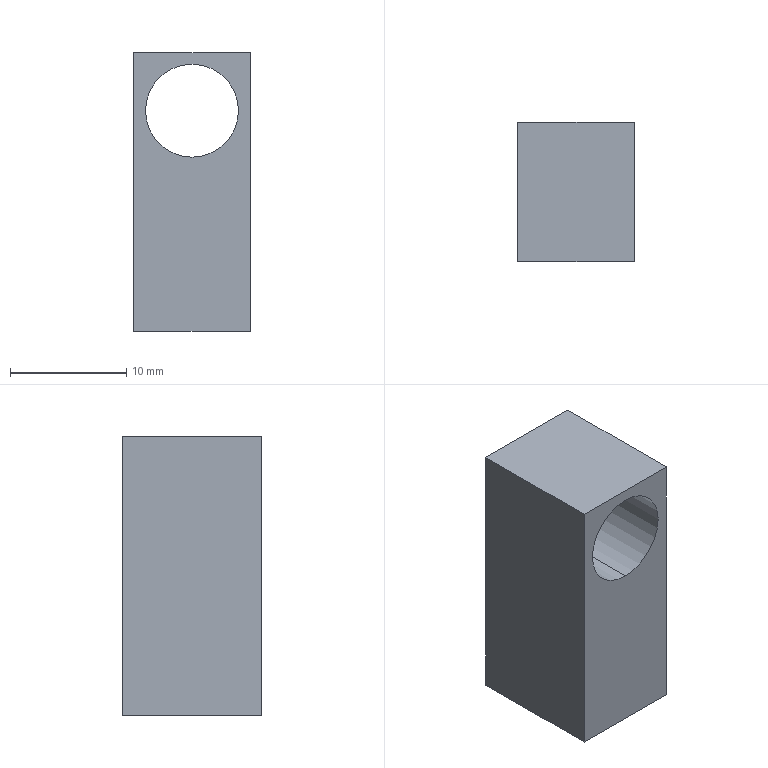Component | SolidWorks | HandlingMechanism-2_A0106-1 | 1 solid | 12 faces | box 10 x 12 x 24 mm | volume 2132 mm3 | plane 6 | cylinder 4 | cone 2 | commonest cylinder face diameters 8 x2 4.2 x2
build123d program:
from build123d import *

# Parameters (mm, degrees)
SKETCH1_W             = 12
SKETCH1_H             = 10
BOSS_EXTRUDE1_DEPTH   = 24
M5_TAPPED_HOLE1_D     = 4.2
M5_TAPPED_HOLE1_DEPTH = 10
M5_TAPPED_HOLE1_TIP   = 1.262
M8X1_0_TAPPED_HOLE1_D = 8


with BuildPart() as part:
    # Sketch1 → Boss-Extrude1 (new body)
    with BuildSketch(Plane.XY):
        Rectangle(SKETCH1_W, SKETCH1_H)
    extrude(amount=BOSS_EXTRUDE1_DEPTH)

    # M5 Tapped Hole1
    with Locations(Plane.XY.offset(24)):
        with Locations((0, 0)):
            Hole(M5_TAPPED_HOLE1_D / 2, depth=M5_TAPPED_HOLE1_DEPTH)
            with Locations((0, 0, -(M5_TAPPED_HOLE1_DEPTH + M5_TAPPED_HOLE1_TIP / 2))):  # 118° drill point
                Cone(0, M5_TAPPED_HOLE1_D / 2, M5_TAPPED_HOLE1_TIP, mode=Mode.SUBTRACT)

    # M8x1.0 Tapped Hole1 (through all)
    with Locations(Plane.ZY.offset(6)):
        with Locations((5, 0)):
            Hole(M8X1_0_TAPPED_HOLE1_D / 2)


solid = part.part

# Placed as in the assembly
solid = solid.moved(Location((80.881, 190.5, 157), (180, 0, -90)))
STEP:
#1=COLOUR_RGB('',0.7922,0.8196,0.9333);
#2=FILL_AREA_STYLE_COLOUR('',#1);
#3=FILL_AREA_STYLE('',(#2));
#4=SURFACE_STYLE_FILL_AREA(#3);
#5=SURFACE_SIDE_STYLE('',(#4));
#6=SURFACE_STYLE_USAGE(.BOTH.,#5);
#7=PRESENTATION_STYLE_ASSIGNMENT((#6));
#8=CARTESIAN_POINT('',(3.184,7.736,6.142));
#9=VERTEX_POINT('',#8);
#10=CARTESIAN_POINT('',(3.184,7.736,5.827));
#11=VERTEX_POINT('',#10);
#12=CARTESIAN_POINT('',(3.184,7.736,5.984));
#13=DIRECTION('',(-0.,-1.,0.));
#14=DIRECTION('',(0.,0.,-1.));
#15=AXIS2_PLACEMENT_3D('',#12,#13,#14);
#16=CIRCLE('',#15,0.1575);
#17=EDGE_CURVE('',#9,#11,#16,.T.);
#18=ORIENTED_EDGE('',*,*,#17,.F.);
#19=CARTESIAN_POINT('',(3.184,7.264,6.142));
#20=VERTEX_POINT('',#19);
#21=CARTESIAN_POINT('',(3.184,7.264,6.142));
#22=DIRECTION('',(-0.,-1.,0.));
#23=VECTOR('',#22,39.37);
#24=LINE('',#21,#23);
#25=EDGE_CURVE('',#9,#20,#24,.T.);
#26=ORIENTED_EDGE('',*,*,#25,.T.);
#27=CARTESIAN_POINT('',(3.184,7.264,5.827));
#28=VERTEX_POINT('',#27);
#29=CARTESIAN_POINT('',(3.184,7.264,5.984));
#30=DIRECTION('',(-0.,-1.,0.));
#31=DIRECTION('',(0.,0.,-1.));
#32=AXIS2_PLACEMENT_3D('',#29,#30,#31);
#33=CIRCLE('',#32,0.1575);
#34=EDGE_CURVE('',#20,#28,#33,.T.);
#35=ORIENTED_EDGE('',*,*,#34,.T.);
#36=CARTESIAN_POINT('',(3.184,7.264,5.827));
#37=DIRECTION('',(-0.,-1.,0.));
#38=VECTOR('',#37,39.37);
#39=LINE('',#36,#38);
#40=EDGE_CURVE('',#11,#28,#39,.T.);
#41=ORIENTED_EDGE('',*,*,#40,.F.);
#42=EDGE_LOOP('',(#18,#26,#35,#41));
#43=FACE_OUTER_BOUND('',#42,.T.);
#44=CARTESIAN_POINT('',(3.184,7.264,5.984));
#45=DIRECTION('',(-0.,-1.,0.));
#46=DIRECTION('',(0.,0.,-1.));
#47=AXIS2_PLACEMENT_3D('',#44,#45,#46);
#48=CYLINDRICAL_SURFACE('',#47,0.1575);
#49=ADVANCED_FACE('',(#43),#48,.F.);
#50=CARTESIAN_POINT('',(3.184,7.417,5.63));
#51=VERTEX_POINT('',#50);
#52=CARTESIAN_POINT('',(3.184,7.583,5.63));
#53=VERTEX_POINT('',#52);
#54=CARTESIAN_POINT('',(3.184,7.5,5.63));
#55=DIRECTION('',(0.,-0.,-1.));
#56=DIRECTION('',(0.,1.,0.));
#57=AXIS2_PLACEMENT_3D('',#54,#55,#56);
#58=CIRCLE('',#57,0.08268);
#59=EDGE_CURVE('',#51,#53,#58,.T.);
#60=ORIENTED_EDGE('',*,*,#59,.F.);
#61=CARTESIAN_POINT('',(3.184,7.417,5.236));
#62=VERTEX_POINT('',#61);
#63=CARTESIAN_POINT('',(3.184,7.417,5.236));
#64=DIRECTION('',(0.,-0.,-1.));
#65=VECTOR('',#64,39.37);
#66=LINE('',#63,#65);
#67=EDGE_CURVE('',#51,#62,#66,.T.);
#68=ORIENTED_EDGE('',*,*,#67,.T.);
#69=CARTESIAN_POINT('',(3.184,7.583,5.236));
#70=VERTEX_POINT('',#69);
#71=CARTESIAN_POINT('',(3.184,7.5,5.236));
#72=DIRECTION('',(0.,-0.,-1.));
#73=DIRECTION('',(0.,1.,0.));
#74=AXIS2_PLACEMENT_3D('',#71,#72,#73);
#75=CIRCLE('',#74,0.08268);
#76=EDGE_CURVE('',#62,#70,#75,.T.);
#77=ORIENTED_EDGE('',*,*,#76,.T.);
#78=CARTESIAN_POINT('',(3.184,7.583,5.236));
#79=DIRECTION('',(0.,-0.,-1.));
#80=VECTOR('',#79,39.37);
#81=LINE('',#78,#80);
#82=EDGE_CURVE('',#53,#70,#81,.T.);
#83=ORIENTED_EDGE('',*,*,#82,.F.);
#84=EDGE_LOOP('',(#60,#68,#77,#83));
#85=FACE_OUTER_BOUND('',#84,.T.);
#86=CARTESIAN_POINT('',(3.184,7.5,5.236));
#87=DIRECTION('',(0.,-0.,-1.));
#88=DIRECTION('',(0.,1.,0.));
#89=AXIS2_PLACEMENT_3D('',#86,#87,#88);
#90=CYLINDRICAL_SURFACE('',#89,0.08268);
#91=ADVANCED_FACE('',(#85),#90,.F.);
#92=CARTESIAN_POINT('',(3.184,7.5,5.68));
#93=VERTEX_POINT('',#92);
#94=CARTESIAN_POINT('',(3.184,7.583,5.63));
#95=DIRECTION('',(0.,0.8572,-0.515));
#96=VECTOR('',#95,39.37);
#97=LINE('',#94,#96);
#98=EDGE_CURVE('',#93,#53,#97,.T.);
#99=ORIENTED_EDGE('',*,*,#98,.F.);
#100=CARTESIAN_POINT('',(3.184,7.417,5.63));
#101=DIRECTION('',(0.,-0.8572,-0.515));
#102=VECTOR('',#101,39.37);
#103=LINE('',#100,#102);
#104=EDGE_CURVE('',#93,#51,#103,.T.);
#105=ORIENTED_EDGE('',*,*,#104,.T.);
#106=ORIENTED_EDGE('',*,*,#59,.T.);
#107=EDGE_LOOP('',(#99,#105,#106));
#108=FACE_OUTER_BOUND('',#107,.T.);
#109=CARTESIAN_POINT('',(3.184,7.5,5.63));
#110=DIRECTION('',(0.,-0.,-1.));
#111=DIRECTION('',(0.,1.,0.));
#112=AXIS2_PLACEMENT_3D('',#109,#110,#111);
#113=CONICAL_SURFACE('',#112,0.08268,1.03);
#114=ADVANCED_FACE('',(#108),#113,.F.);
#115=CARTESIAN_POINT('',(3.184,7.736,5.984));
#116=DIRECTION('',(-0.,-1.,0.));
#117=DIRECTION('',(0.,0.,-1.));
#118=AXIS2_PLACEMENT_3D('',#115,#116,#117);
#119=CIRCLE('',#118,0.1575);
#120=EDGE_CURVE('',#11,#9,#119,.T.);
#121=ORIENTED_EDGE('',*,*,#120,.T.);
#122=ORIENTED_EDGE('',*,*,#17,.T.);
#123=EDGE_LOOP('',(#121,#122));
#124=FACE_BOUND('',#123,.T.);
#125=CARTESIAN_POINT('',(2.987,7.736,6.181));
#126=VERTEX_POINT('',#125);
#127=CARTESIAN_POINT('',(3.381,7.736,6.181));
#128=VERTEX_POINT('',#127);
#129=CARTESIAN_POINT('',(3.381,7.736,6.181));
#130=DIRECTION('',(1.,-0.,0.));
#131=VECTOR('',#130,39.37);
#132=LINE('',#129,#131);
#133=EDGE_CURVE('',#126,#128,#132,.T.);
#134=ORIENTED_EDGE('',*,*,#133,.T.);
#135=CARTESIAN_POINT('',(3.381,7.736,5.236));
#136=VERTEX_POINT('',#135);
#137=CARTESIAN_POINT('',(3.381,7.736,5.236));
#138=DIRECTION('',(-0.,0.,1.));
#139=VECTOR('',#138,39.37);
#140=LINE('',#137,#139);
#141=EDGE_CURVE('',#136,#128,#140,.T.);
#142=ORIENTED_EDGE('',*,*,#141,.F.);
#143=CARTESIAN_POINT('',(2.987,7.736,5.236));
#144=VERTEX_POINT('',#143);
#145=CARTESIAN_POINT('',(3.381,7.736,5.236));
#146=DIRECTION('',(1.,-0.,0.));
#147=VECTOR('',#146,39.37);
#148=LINE('',#145,#147);
#149=EDGE_CURVE('',#144,#136,#148,.T.);
#150=ORIENTED_EDGE('',*,*,#149,.F.);
#151=CARTESIAN_POINT('',(2.987,7.736,5.236));
#152=DIRECTION('',(-0.,0.,1.));
#153=VECTOR('',#152,39.37);
#154=LINE('',#151,#153);
#155=EDGE_CURVE('',#144,#126,#154,.T.);
#156=ORIENTED_EDGE('',*,*,#155,.T.);
#157=EDGE_LOOP('',(#134,#142,#150,#156));
#158=FACE_OUTER_BOUND('',#157,.T.);
#159=CARTESIAN_POINT('',(3.381,7.736,5.236));
#160=DIRECTION('',(-0.,-1.,0.));
#161=DIRECTION('',(-1.,0.,-0.));
#162=AXIS2_PLACEMENT_3D('',#159,#160,#161);
#163=PLANE('',#162);
#164=ADVANCED_FACE('',(#124,#158),#163,.F.);
#165=CARTESIAN_POINT('',(3.381,7.264,6.181));
#166=VERTEX_POINT('',#165);
#167=CARTESIAN_POINT('',(3.381,7.264,6.181));
#168=DIRECTION('',(-0.,-1.,0.));
#169=VECTOR('',#168,39.37);
#170=LINE('',#167,#169);
#171=EDGE_CURVE('',#128,#166,#170,.T.);
#172=ORIENTED_EDGE('',*,*,#171,.T.);
#173=CARTESIAN_POINT('',(3.381,7.264,5.236));
#174=VERTEX_POINT('',#173);
#175=CARTESIAN_POINT('',(3.381,7.264,5.236));
#176=DIRECTION('',(-0.,0.,1.));
#177=VECTOR('',#176,39.37);
#178=LINE('',#175,#177);
#179=EDGE_CURVE('',#174,#166,#178,.T.);
#180=ORIENTED_EDGE('',*,*,#179,.F.);
#181=CARTESIAN_POINT('',(3.381,7.264,5.236));
#182=DIRECTION('',(-0.,-1.,0.));
#183=VECTOR('',#182,39.37);
#184=LINE('',#181,#183);
#185=EDGE_CURVE('',#136,#174,#184,.T.);
#186=ORIENTED_EDGE('',*,*,#185,.F.);
#187=ORIENTED_EDGE('',*,*,#141,.T.);
#188=EDGE_LOOP('',(#172,#180,#186,#187));
#189=FACE_OUTER_BOUND('',#188,.T.);
#190=CARTESIAN_POINT('',(3.381,7.264,5.236));
#191=DIRECTION('',(-1.,0.,-0.));
#192=DIRECTION('',(-0.,0.,1.));
#193=AXIS2_PLACEMENT_3D('',#190,#191,#192);
#194=PLANE('',#193);
#195=ADVANCED_FACE('',(#189),#194,.F.);
#196=CARTESIAN_POINT('',(3.184,7.264,5.984));
#197=DIRECTION('',(-0.,-1.,0.));
#198=DIRECTION('',(0.,0.,-1.));
#199=AXIS2_PLACEMENT_3D('',#196,#197,#198);
#200=CIRCLE('',#199,0.1575);
#201=EDGE_CURVE('',#28,#20,#200,.T.);
#202=ORIENTED_EDGE('',*,*,#201,.F.);
#203=ORIENTED_EDGE('',*,*,#34,.F.);
#204=EDGE_LOOP('',(#202,#203));
#205=FACE_BOUND('',#204,.T.);
#206=CARTESIAN_POINT('',(2.987,7.264,6.181));
#207=VERTEX_POINT('',#206);
#208=CARTESIAN_POINT('',(3.381,7.264,6.181));
#209=DIRECTION('',(-1.,0.,-0.));
#210=VECTOR('',#209,39.37);
#211=LINE('',#208,#210);
#212=EDGE_CURVE('',#166,#207,#211,.T.);
#213=ORIENTED_EDGE('',*,*,#212,.T.);
#214=CARTESIAN_POINT('',(2.987,7.264,5.236));
#215=VERTEX_POINT('',#214);
#216=CARTESIAN_POINT('',(2.987,7.264,5.236));
#217=DIRECTION('',(-0.,0.,1.));
#218=VECTOR('',#217,39.37);
#219=LINE('',#216,#218);
#220=EDGE_CURVE('',#215,#207,#219,.T.);
#221=ORIENTED_EDGE('',*,*,#220,.F.);
#222=CARTESIAN_POINT('',(3.381,7.264,5.236));
#223=DIRECTION('',(-1.,0.,-0.));
#224=VECTOR('',#223,39.37);
#225=LINE('',#222,#224);
#226=EDGE_CURVE('',#174,#215,#225,.T.);
#227=ORIENTED_EDGE('',*,*,#226,.F.);
#228=ORIENTED_EDGE('',*,*,#179,.T.);
#229=EDGE_LOOP('',(#213,#221,#227,#228));
#230=FACE_OUTER_BOUND('',#229,.T.);
#231=CARTESIAN_POINT('',(3.381,7.264,5.236));
#232=DIRECTION('',(0.,1.,-0.));
#233=DIRECTION('',(-0.,0.,1.));
#234=AXIS2_PLACEMENT_3D('',#231,#232,#233);
#235=PLANE('',#234);
#236=ADVANCED_FACE('',(#205,#230),#235,.F.);
#237=CARTESIAN_POINT('',(2.987,7.264,6.181));
#238=DIRECTION('',(0.,1.,-0.));
#239=VECTOR('',#238,39.37);
#240=LINE('',#237,#239);
#241=EDGE_CURVE('',#207,#126,#240,.T.);
#242=ORIENTED_EDGE('',*,*,#241,.T.);
#243=ORIENTED_EDGE('',*,*,#155,.F.);
#244=CARTESIAN_POINT('',(2.987,7.264,5.236));
#245=DIRECTION('',(0.,1.,-0.));
#246=VECTOR('',#245,39.37);
#247=LINE('',#244,#246);
#248=EDGE_CURVE('',#215,#144,#247,.T.);
#249=ORIENTED_EDGE('',*,*,#248,.F.);
#250=ORIENTED_EDGE('',*,*,#220,.T.);
#251=EDGE_LOOP('',(#242,#243,#249,#250));
#252=FACE_OUTER_BOUND('',#251,.T.);
#253=CARTESIAN_POINT('',(2.987,7.264,5.236));
#254=DIRECTION('',(1.,-0.,0.));
#255=DIRECTION('',(0.,-0.,-1.));
#256=AXIS2_PLACEMENT_3D('',#253,#254,#255);
#257=PLANE('',#256);
#258=ADVANCED_FACE('',(#252),#257,.F.);
#259=CARTESIAN_POINT('',(3.184,7.5,5.236));
#260=DIRECTION('',(0.,-0.,-1.));
#261=DIRECTION('',(0.,1.,0.));
#262=AXIS2_PLACEMENT_3D('',#259,#260,#261);
#263=CIRCLE('',#262,0.08268);
#264=EDGE_CURVE('',#70,#62,#263,.T.);
#265=ORIENTED_EDGE('',*,*,#264,.F.);
#266=ORIENTED_EDGE('',*,*,#76,.F.);
#267=EDGE_LOOP('',(#265,#266));
#268=FACE_BOUND('',#267,.T.);
#269=ORIENTED_EDGE('',*,*,#149,.T.);
#270=ORIENTED_EDGE('',*,*,#185,.T.);
#271=ORIENTED_EDGE('',*,*,#226,.T.);
#272=ORIENTED_EDGE('',*,*,#248,.T.);
#273=EDGE_LOOP('',(#269,#270,#271,#272));
#274=FACE_OUTER_BOUND('',#273,.T.);
#275=CARTESIAN_POINT('',(3.184,7.5,5.236));
#276=DIRECTION('',(0.,-0.,-1.));
#277=DIRECTION('',(0.,1.,-0.));
#278=AXIS2_PLACEMENT_3D('',#275,#276,#277);
#279=PLANE('',#278);
#280=ADVANCED_FACE('',(#268,#274),#279,.T.);
#281=ORIENTED_EDGE('',*,*,#133,.F.);
#282=ORIENTED_EDGE('',*,*,#241,.F.);
#283=ORIENTED_EDGE('',*,*,#212,.F.);
#284=ORIENTED_EDGE('',*,*,#171,.F.);
#285=EDGE_LOOP('',(#281,#282,#283,#284));
#286=FACE_OUTER_BOUND('',#285,.T.);
#287=CARTESIAN_POINT('',(3.184,7.5,6.181));
#288=DIRECTION('',(0.,-0.,-1.));
#289=DIRECTION('',(0.,1.,-0.));
#290=AXIS2_PLACEMENT_3D('',#287,#288,#289);
#291=PLANE('',#290);
#292=ADVANCED_FACE('',(#286),#291,.F.);
#293=ORIENTED_EDGE('',*,*,#104,.F.);
#294=ORIENTED_EDGE('',*,*,#98,.T.);
#295=CARTESIAN_POINT('',(3.184,7.5,5.63));
#296=DIRECTION('',(0.,-0.,-1.));
#297=DIRECTION('',(0.,1.,0.));
#298=AXIS2_PLACEMENT_3D('',#295,#296,#297);
#299=CIRCLE('',#298,0.08268);
#300=EDGE_CURVE('',#53,#51,#299,.T.);
#301=ORIENTED_EDGE('',*,*,#300,.T.);
#302=EDGE_LOOP('',(#293,#294,#301));
#303=FACE_OUTER_BOUND('',#302,.T.);
#304=CARTESIAN_POINT('',(3.184,7.5,5.63));
#305=DIRECTION('',(0.,-0.,-1.));
#306=DIRECTION('',(0.,1.,0.));
#307=AXIS2_PLACEMENT_3D('',#304,#305,#306);
#308=CONICAL_SURFACE('',#307,0.08268,1.03);
#309=ADVANCED_FACE('',(#303),#308,.F.);
#310=ORIENTED_EDGE('',*,*,#67,.F.);
#311=ORIENTED_EDGE('',*,*,#300,.F.);
#312=ORIENTED_EDGE('',*,*,#82,.T.);
#313=ORIENTED_EDGE('',*,*,#264,.T.);
#314=EDGE_LOOP('',(#310,#311,#312,#313));
#315=FACE_OUTER_BOUND('',#314,.T.);
#316=CARTESIAN_POINT('',(3.184,7.5,5.236));
#317=DIRECTION('',(0.,-0.,-1.));
#318=DIRECTION('',(0.,1.,0.));
#319=AXIS2_PLACEMENT_3D('',#316,#317,#318);
#320=CYLINDRICAL_SURFACE('',#319,0.08268);
#321=ADVANCED_FACE('',(#315),#320,.F.);
#322=ORIENTED_EDGE('',*,*,#25,.F.);
#323=ORIENTED_EDGE('',*,*,#120,.F.);
#324=ORIENTED_EDGE('',*,*,#40,.T.);
#325=ORIENTED_EDGE('',*,*,#201,.T.);
#326=EDGE_LOOP('',(#322,#323,#324,#325));
#327=FACE_OUTER_BOUND('',#326,.T.);
#328=CARTESIAN_POINT('',(3.184,7.264,5.984));
#329=DIRECTION('',(-0.,-1.,0.));
#330=DIRECTION('',(0.,0.,-1.));
#331=AXIS2_PLACEMENT_3D('',#328,#329,#330);
#332=CYLINDRICAL_SURFACE('',#331,0.1575);
#333=ADVANCED_FACE('',(#327),#332,.F.);
#334=CLOSED_SHELL('',(#49,#91,#114,#164,#195,#236,#258,#280,#292,#309,#321,#333));
#335=MANIFOLD_SOLID_BREP('',#334);
#336=STYLED_ITEM('',(#7),#335);
#337=(LENGTH_UNIT()NAMED_UNIT(*)SI_UNIT($,.METRE.));
#338=LENGTH_MEASURE_WITH_UNIT(LENGTH_MEASURE(0.0254),#337);
#339=DIMENSIONAL_EXPONENTS(1.,0.,0.,0.,0.,0.,0.);
#340=(CONVERSION_BASED_UNIT('',#338)LENGTH_UNIT()NAMED_UNIT(#339));
#341=UNCERTAINTY_MEASURE_WITH_UNIT(LENGTH_MEASURE(0.00001),#340,'','');
#342=(NAMED_UNIT(*)PLANE_ANGLE_UNIT()SI_UNIT($,.RADIAN.));
#343=(NAMED_UNIT(*)SI_UNIT($,.STERADIAN.)SOLID_ANGLE_UNIT());
#344=(GEOMETRIC_REPRESENTATION_CONTEXT(3)GLOBAL_UNCERTAINTY_ASSIGNED_CONTEXT((#341))GLOBAL_UNIT_ASSIGNED_CONTEXT((#340,#342,#343))REPRESENTATION_CONTEXT('',''));
#345=MECHANICAL_DESIGN_GEOMETRIC_PRESENTATION_REPRESENTATION('',(#336),#344);
#346=PRESENTATION_LAYER_ASSIGNMENT('','',(#336));
#347=CARTESIAN_POINT('',(0.,0.,0.));
#348=DIRECTION('',(0.,0.,1.));
#349=DIRECTION('',(1.,0.,0.));
#350=AXIS2_PLACEMENT_3D('',#347,#348,#349);
#351=(LENGTH_UNIT()NAMED_UNIT(*)SI_UNIT($,.METRE.));
#352=LENGTH_MEASURE_WITH_UNIT(LENGTH_MEASURE(0.0254),#351);
#353=DIMENSIONAL_EXPONENTS(1.,0.,0.,0.,0.,0.,0.);
#354=(CONVERSION_BASED_UNIT('',#352)LENGTH_UNIT()NAMED_UNIT(#353));
#355=UNCERTAINTY_MEASURE_WITH_UNIT(LENGTH_MEASURE(0.00001),#354,'','');
#356=(NAMED_UNIT(*)PLANE_ANGLE_UNIT()SI_UNIT($,.RADIAN.));
#357=(NAMED_UNIT(*)SI_UNIT($,.STERADIAN.)SOLID_ANGLE_UNIT());
#358=(GEOMETRIC_REPRESENTATION_CONTEXT(3)GLOBAL_UNCERTAINTY_ASSIGNED_CONTEXT((#355))GLOBAL_UNIT_ASSIGNED_CONTEXT((#354,#356,#357))REPRESENTATION_CONTEXT('',''));
#359=ADVANCED_BREP_SHAPE_REPRESENTATION('',(#335,#350),#358);